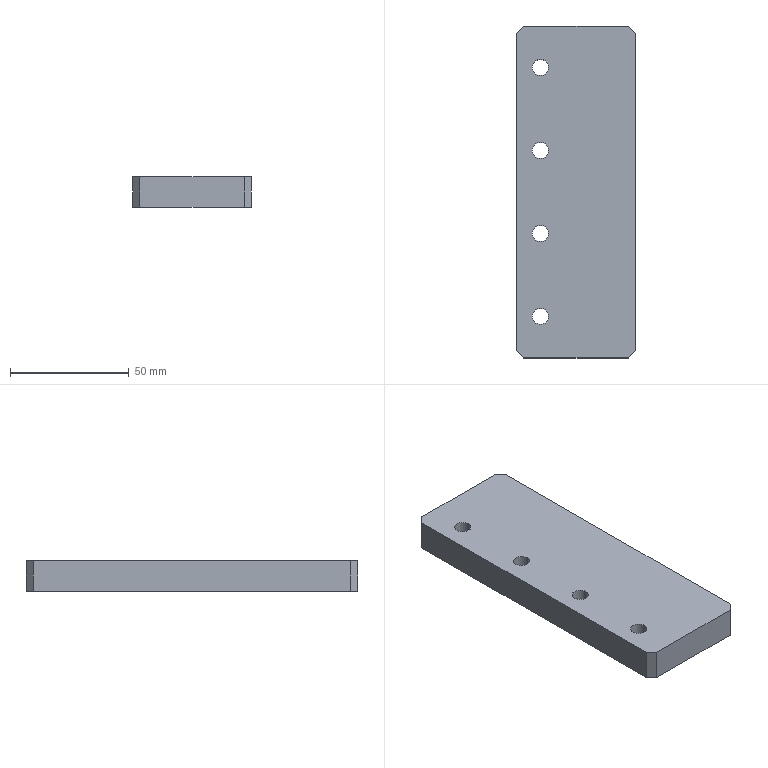Component | SolidWorks | STE21014.01-41-1 | 1 solid | 18 faces | box 50 x 140 x 13 mm | volume 88878 mm3 | plane 10 | cylinder 8 | commonest cylinder face diameters 6.8 x8 | material Q235
build123d program:
from build123d import *

# Parameters (mm, degrees)
SKETCH1_W           = 140
SKETCH1_H           = 50
BOSS_EXTRUDE1_DEPTH = 13
M8_TAPPED_HOLE1_D   = 6.8
CHAMFER1_SIZE       = 3


with BuildPart() as part:
    # Sketch1 → Boss-Extrude1 (new body)
    with BuildSketch(Plane(origin=(0, 0, 0), x_dir=(1, 0, 0), z_dir=(0, 1, 0))):
        Rectangle(SKETCH1_W, SKETCH1_H)
    extrude(amount=BOSS_EXTRUDE1_DEPTH)

    # M8 Tapped Hole1 (through all)
    with Locations(Plane(origin=(0, 13, 0), x_dir=(1, 0, 0), z_dir=(0, 1, 0))):
        with Locations((-52.5, -15), (-17.5, -15), (17.5, -15), (52.5, -15)):
            Hole(M8_TAPPED_HOLE1_D / 2)

    # Chamfer1
    chamfer1_edges = [part.edges().sort_by_distance(p)[0] for p in [
        (-70, 6.5, -25),
        (70, 6.5, -25),
        (70, 6.5, 25),
        (-70, 6.5, 25),
    ]]
    chamfer(chamfer1_edges, length=CHAMFER1_SIZE)


solid = part.part

# Placed as in the assembly
solid = solid.moved(Location((615, 550, -623), (90, -90, 0)))
STEP:
#1=COLOUR_RGB('',0.7922,0.8196,0.9333);
#2=FILL_AREA_STYLE_COLOUR('',#1);
#3=FILL_AREA_STYLE('',(#2));
#4=SURFACE_STYLE_FILL_AREA(#3);
#5=SURFACE_SIDE_STYLE('',(#4));
#6=SURFACE_STYLE_USAGE(.BOTH.,#5);
#7=PRESENTATION_STYLE_ASSIGNMENT((#6));
#8=CARTESIAN_POINT('',(23.756,23.72,-24.528));
#9=VERTEX_POINT('',#8);
#10=CARTESIAN_POINT('',(23.488,23.72,-24.528));
#11=VERTEX_POINT('',#10);
#12=CARTESIAN_POINT('',(23.622,23.72,-24.528));
#13=DIRECTION('',(0.,-0.,1.));
#14=DIRECTION('',(-1.,0.,0.));
#15=AXIS2_PLACEMENT_3D('',#12,#13,#14);
#16=CIRCLE('',#15,0.1339);
#17=EDGE_CURVE('',#9,#11,#16,.T.);
#18=ORIENTED_EDGE('',*,*,#17,.F.);
#19=CARTESIAN_POINT('',(23.756,23.72,-24.016));
#20=VERTEX_POINT('',#19);
#21=CARTESIAN_POINT('',(23.756,23.72,-24.016));
#22=DIRECTION('',(0.,-0.,1.));
#23=VECTOR('',#22,39.37);
#24=LINE('',#21,#23);
#25=EDGE_CURVE('',#9,#20,#24,.T.);
#26=ORIENTED_EDGE('',*,*,#25,.T.);
#27=CARTESIAN_POINT('',(23.488,23.72,-24.016));
#28=VERTEX_POINT('',#27);
#29=CARTESIAN_POINT('',(23.622,23.72,-24.016));
#30=DIRECTION('',(0.,-0.,1.));
#31=DIRECTION('',(-1.,0.,0.));
#32=AXIS2_PLACEMENT_3D('',#29,#30,#31);
#33=CIRCLE('',#32,0.1339);
#34=EDGE_CURVE('',#20,#28,#33,.T.);
#35=ORIENTED_EDGE('',*,*,#34,.T.);
#36=CARTESIAN_POINT('',(23.488,23.72,-24.016));
#37=DIRECTION('',(0.,-0.,1.));
#38=VECTOR('',#37,39.37);
#39=LINE('',#36,#38);
#40=EDGE_CURVE('',#11,#28,#39,.T.);
#41=ORIENTED_EDGE('',*,*,#40,.F.);
#42=EDGE_LOOP('',(#18,#26,#35,#41));
#43=FACE_OUTER_BOUND('',#42,.T.);
#44=CARTESIAN_POINT('',(23.622,23.72,-24.016));
#45=DIRECTION('',(0.,-0.,1.));
#46=DIRECTION('',(-1.,0.,0.));
#47=AXIS2_PLACEMENT_3D('',#44,#45,#46);
#48=CYLINDRICAL_SURFACE('',#47,0.1339);
#49=ADVANCED_FACE('',(#43),#48,.F.);
#50=CARTESIAN_POINT('',(23.756,22.343,-24.528));
#51=VERTEX_POINT('',#50);
#52=CARTESIAN_POINT('',(23.488,22.343,-24.528));
#53=VERTEX_POINT('',#52);
#54=CARTESIAN_POINT('',(23.622,22.343,-24.528));
#55=DIRECTION('',(0.,-0.,1.));
#56=DIRECTION('',(-1.,0.,0.));
#57=AXIS2_PLACEMENT_3D('',#54,#55,#56);
#58=CIRCLE('',#57,0.1339);
#59=EDGE_CURVE('',#51,#53,#58,.T.);
#60=ORIENTED_EDGE('',*,*,#59,.F.);
#61=CARTESIAN_POINT('',(23.756,22.343,-24.016));
#62=VERTEX_POINT('',#61);
#63=CARTESIAN_POINT('',(23.756,22.343,-24.016));
#64=DIRECTION('',(0.,-0.,1.));
#65=VECTOR('',#64,39.37);
#66=LINE('',#63,#65);
#67=EDGE_CURVE('',#51,#62,#66,.T.);
#68=ORIENTED_EDGE('',*,*,#67,.T.);
#69=CARTESIAN_POINT('',(23.488,22.343,-24.016));
#70=VERTEX_POINT('',#69);
#71=CARTESIAN_POINT('',(23.622,22.343,-24.016));
#72=DIRECTION('',(0.,-0.,1.));
#73=DIRECTION('',(-1.,0.,0.));
#74=AXIS2_PLACEMENT_3D('',#71,#72,#73);
#75=CIRCLE('',#74,0.1339);
#76=EDGE_CURVE('',#62,#70,#75,.T.);
#77=ORIENTED_EDGE('',*,*,#76,.T.);
#78=CARTESIAN_POINT('',(23.488,22.343,-24.016));
#79=DIRECTION('',(0.,-0.,1.));
#80=VECTOR('',#79,39.37);
#81=LINE('',#78,#80);
#82=EDGE_CURVE('',#53,#70,#81,.T.);
#83=ORIENTED_EDGE('',*,*,#82,.F.);
#84=EDGE_LOOP('',(#60,#68,#77,#83));
#85=FACE_OUTER_BOUND('',#84,.T.);
#86=CARTESIAN_POINT('',(23.622,22.343,-24.016));
#87=DIRECTION('',(0.,-0.,1.));
#88=DIRECTION('',(-1.,0.,0.));
#89=AXIS2_PLACEMENT_3D('',#86,#87,#88);
#90=CYLINDRICAL_SURFACE('',#89,0.1339);
#91=ADVANCED_FACE('',(#85),#90,.F.);
#92=CARTESIAN_POINT('',(23.756,20.965,-24.528));
#93=VERTEX_POINT('',#92);
#94=CARTESIAN_POINT('',(23.488,20.965,-24.528));
#95=VERTEX_POINT('',#94);
#96=CARTESIAN_POINT('',(23.622,20.965,-24.528));
#97=DIRECTION('',(0.,-0.,1.));
#98=DIRECTION('',(-1.,0.,0.));
#99=AXIS2_PLACEMENT_3D('',#96,#97,#98);
#100=CIRCLE('',#99,0.1339);
#101=EDGE_CURVE('',#93,#95,#100,.T.);
#102=ORIENTED_EDGE('',*,*,#101,.F.);
#103=CARTESIAN_POINT('',(23.756,20.965,-24.016));
#104=VERTEX_POINT('',#103);
#105=CARTESIAN_POINT('',(23.756,20.965,-24.016));
#106=DIRECTION('',(0.,-0.,1.));
#107=VECTOR('',#106,39.37);
#108=LINE('',#105,#107);
#109=EDGE_CURVE('',#93,#104,#108,.T.);
#110=ORIENTED_EDGE('',*,*,#109,.T.);
#111=CARTESIAN_POINT('',(23.488,20.965,-24.016));
#112=VERTEX_POINT('',#111);
#113=CARTESIAN_POINT('',(23.622,20.965,-24.016));
#114=DIRECTION('',(0.,-0.,1.));
#115=DIRECTION('',(-1.,0.,0.));
#116=AXIS2_PLACEMENT_3D('',#113,#114,#115);
#117=CIRCLE('',#116,0.1339);
#118=EDGE_CURVE('',#104,#112,#117,.T.);
#119=ORIENTED_EDGE('',*,*,#118,.T.);
#120=CARTESIAN_POINT('',(23.488,20.965,-24.016));
#121=DIRECTION('',(0.,-0.,1.));
#122=VECTOR('',#121,39.37);
#123=LINE('',#120,#122);
#124=EDGE_CURVE('',#95,#112,#123,.T.);
#125=ORIENTED_EDGE('',*,*,#124,.F.);
#126=EDGE_LOOP('',(#102,#110,#119,#125));
#127=FACE_OUTER_BOUND('',#126,.T.);
#128=CARTESIAN_POINT('',(23.622,20.965,-24.016));
#129=DIRECTION('',(0.,-0.,1.));
#130=DIRECTION('',(-1.,0.,0.));
#131=AXIS2_PLACEMENT_3D('',#128,#129,#130);
#132=CYLINDRICAL_SURFACE('',#131,0.1339);
#133=ADVANCED_FACE('',(#127),#132,.F.);
#134=CARTESIAN_POINT('',(23.756,19.587,-24.528));
#135=VERTEX_POINT('',#134);
#136=CARTESIAN_POINT('',(23.488,19.587,-24.528));
#137=VERTEX_POINT('',#136);
#138=CARTESIAN_POINT('',(23.622,19.587,-24.528));
#139=DIRECTION('',(0.,-0.,1.));
#140=DIRECTION('',(-1.,0.,0.));
#141=AXIS2_PLACEMENT_3D('',#138,#139,#140);
#142=CIRCLE('',#141,0.1339);
#143=EDGE_CURVE('',#135,#137,#142,.T.);
#144=ORIENTED_EDGE('',*,*,#143,.F.);
#145=CARTESIAN_POINT('',(23.756,19.587,-24.016));
#146=VERTEX_POINT('',#145);
#147=CARTESIAN_POINT('',(23.756,19.587,-24.016));
#148=DIRECTION('',(0.,-0.,1.));
#149=VECTOR('',#148,39.37);
#150=LINE('',#147,#149);
#151=EDGE_CURVE('',#135,#146,#150,.T.);
#152=ORIENTED_EDGE('',*,*,#151,.T.);
#153=CARTESIAN_POINT('',(23.488,19.587,-24.016));
#154=VERTEX_POINT('',#153);
#155=CARTESIAN_POINT('',(23.622,19.587,-24.016));
#156=DIRECTION('',(0.,-0.,1.));
#157=DIRECTION('',(-1.,0.,0.));
#158=AXIS2_PLACEMENT_3D('',#155,#156,#157);
#159=CIRCLE('',#158,0.1339);
#160=EDGE_CURVE('',#146,#154,#159,.T.);
#161=ORIENTED_EDGE('',*,*,#160,.T.);
#162=CARTESIAN_POINT('',(23.488,19.587,-24.016));
#163=DIRECTION('',(0.,-0.,1.));
#164=VECTOR('',#163,39.37);
#165=LINE('',#162,#164);
#166=EDGE_CURVE('',#137,#154,#165,.T.);
#167=ORIENTED_EDGE('',*,*,#166,.F.);
#168=EDGE_LOOP('',(#144,#152,#161,#167));
#169=FACE_OUTER_BOUND('',#168,.T.);
#170=CARTESIAN_POINT('',(23.622,19.587,-24.016));
#171=DIRECTION('',(0.,-0.,1.));
#172=DIRECTION('',(-1.,0.,0.));
#173=AXIS2_PLACEMENT_3D('',#170,#171,#172);
#174=CYLINDRICAL_SURFACE('',#173,0.1339);
#175=ADVANCED_FACE('',(#169),#174,.F.);
#176=CARTESIAN_POINT('',(25.079,24.409,-24.016));
#177=VERTEX_POINT('',#176);
#178=CARTESIAN_POINT('',(23.346,24.409,-24.016));
#179=VERTEX_POINT('',#178);
#180=CARTESIAN_POINT('',(23.228,24.409,-24.016));
#181=DIRECTION('',(-1.,0.,0.));
#182=VECTOR('',#181,39.37);
#183=LINE('',#180,#182);
#184=EDGE_CURVE('',#177,#179,#183,.T.);
#185=ORIENTED_EDGE('',*,*,#184,.F.);
#186=CARTESIAN_POINT('',(25.079,24.409,-24.528));
#187=VERTEX_POINT('',#186);
#188=CARTESIAN_POINT('',(25.079,24.409,-24.016));
#189=DIRECTION('',(-0.,0.,-1.));
#190=VECTOR('',#189,39.37);
#191=LINE('',#188,#190);
#192=EDGE_CURVE('',#177,#187,#191,.T.);
#193=ORIENTED_EDGE('',*,*,#192,.T.);
#194=CARTESIAN_POINT('',(23.346,24.409,-24.528));
#195=VERTEX_POINT('',#194);
#196=CARTESIAN_POINT('',(23.228,24.409,-24.528));
#197=DIRECTION('',(-1.,0.,0.));
#198=VECTOR('',#197,39.37);
#199=LINE('',#196,#198);
#200=EDGE_CURVE('',#187,#195,#199,.T.);
#201=ORIENTED_EDGE('',*,*,#200,.T.);
#202=CARTESIAN_POINT('',(23.346,24.409,-24.016));
#203=DIRECTION('',(0.,-0.,1.));
#204=VECTOR('',#203,39.37);
#205=LINE('',#202,#204);
#206=EDGE_CURVE('',#195,#179,#205,.T.);
#207=ORIENTED_EDGE('',*,*,#206,.T.);
#208=EDGE_LOOP('',(#185,#193,#201,#207));
#209=FACE_OUTER_BOUND('',#208,.T.);
#210=CARTESIAN_POINT('',(23.228,24.409,-24.016));
#211=DIRECTION('',(-0.,-1.,-0.));
#212=DIRECTION('',(1.,-0.,-0.));
#213=AXIS2_PLACEMENT_3D('',#210,#211,#212);
#214=PLANE('',#213);
#215=ADVANCED_FACE('',(#209),#214,.F.);
#216=CARTESIAN_POINT('',(23.228,24.291,-24.528));
#217=VERTEX_POINT('',#216);
#218=CARTESIAN_POINT('',(23.228,19.016,-24.528));
#219=VERTEX_POINT('',#218);
#220=CARTESIAN_POINT('',(23.228,18.898,-24.528));
#221=DIRECTION('',(0.,-1.,-0.));
#222=VECTOR('',#221,39.37);
#223=LINE('',#220,#222);
#224=EDGE_CURVE('',#217,#219,#223,.T.);
#225=ORIENTED_EDGE('',*,*,#224,.T.);
#226=CARTESIAN_POINT('',(23.228,19.016,-24.016));
#227=VERTEX_POINT('',#226);
#228=CARTESIAN_POINT('',(23.228,19.016,-24.016));
#229=DIRECTION('',(0.,-0.,1.));
#230=VECTOR('',#229,39.37);
#231=LINE('',#228,#230);
#232=EDGE_CURVE('',#219,#227,#231,.T.);
#233=ORIENTED_EDGE('',*,*,#232,.T.);
#234=CARTESIAN_POINT('',(23.228,24.291,-24.016));
#235=VERTEX_POINT('',#234);
#236=CARTESIAN_POINT('',(23.228,18.898,-24.016));
#237=DIRECTION('',(0.,-1.,-0.));
#238=VECTOR('',#237,39.37);
#239=LINE('',#236,#238);
#240=EDGE_CURVE('',#235,#227,#239,.T.);
#241=ORIENTED_EDGE('',*,*,#240,.F.);
#242=CARTESIAN_POINT('',(23.228,24.291,-24.016));
#243=DIRECTION('',(-0.,0.,-1.));
#244=VECTOR('',#243,39.37);
#245=LINE('',#242,#244);
#246=EDGE_CURVE('',#235,#217,#245,.T.);
#247=ORIENTED_EDGE('',*,*,#246,.T.);
#248=EDGE_LOOP('',(#225,#233,#241,#247));
#249=FACE_OUTER_BOUND('',#248,.T.);
#250=CARTESIAN_POINT('',(23.228,18.898,-24.016));
#251=DIRECTION('',(1.,0.,-0.));
#252=DIRECTION('',(-0.,1.,0.));
#253=AXIS2_PLACEMENT_3D('',#250,#251,#252);
#254=PLANE('',#253);
#255=ADVANCED_FACE('',(#249),#254,.F.);
#256=CARTESIAN_POINT('',(23.346,18.898,-24.016));
#257=VERTEX_POINT('',#256);
#258=CARTESIAN_POINT('',(25.079,18.898,-24.016));
#259=VERTEX_POINT('',#258);
#260=CARTESIAN_POINT('',(23.228,18.898,-24.016));
#261=DIRECTION('',(1.,-0.,-0.));
#262=VECTOR('',#261,39.37);
#263=LINE('',#260,#262);
#264=EDGE_CURVE('',#257,#259,#263,.T.);
#265=ORIENTED_EDGE('',*,*,#264,.F.);
#266=CARTESIAN_POINT('',(23.346,18.898,-24.528));
#267=VERTEX_POINT('',#266);
#268=CARTESIAN_POINT('',(23.346,18.898,-24.016));
#269=DIRECTION('',(-0.,0.,-1.));
#270=VECTOR('',#269,39.37);
#271=LINE('',#268,#270);
#272=EDGE_CURVE('',#257,#267,#271,.T.);
#273=ORIENTED_EDGE('',*,*,#272,.T.);
#274=CARTESIAN_POINT('',(25.079,18.898,-24.528));
#275=VERTEX_POINT('',#274);
#276=CARTESIAN_POINT('',(23.228,18.898,-24.528));
#277=DIRECTION('',(1.,-0.,-0.));
#278=VECTOR('',#277,39.37);
#279=LINE('',#276,#278);
#280=EDGE_CURVE('',#267,#275,#279,.T.);
#281=ORIENTED_EDGE('',*,*,#280,.T.);
#282=CARTESIAN_POINT('',(25.079,18.898,-24.016));
#283=DIRECTION('',(0.,-0.,1.));
#284=VECTOR('',#283,39.37);
#285=LINE('',#282,#284);
#286=EDGE_CURVE('',#275,#259,#285,.T.);
#287=ORIENTED_EDGE('',*,*,#286,.T.);
#288=EDGE_LOOP('',(#265,#273,#281,#287));
#289=FACE_OUTER_BOUND('',#288,.T.);
#290=CARTESIAN_POINT('',(23.228,18.898,-24.016));
#291=DIRECTION('',(0.,1.,0.));
#292=DIRECTION('',(-1.,0.,0.));
#293=AXIS2_PLACEMENT_3D('',#290,#291,#292);
#294=PLANE('',#293);
#295=ADVANCED_FACE('',(#289),#294,.F.);
#296=CARTESIAN_POINT('',(25.197,19.016,-24.016));
#297=VERTEX_POINT('',#296);
#298=CARTESIAN_POINT('',(25.197,24.291,-24.016));
#299=VERTEX_POINT('',#298);
#300=CARTESIAN_POINT('',(25.197,18.898,-24.016));
#301=DIRECTION('',(-0.,1.,0.));
#302=VECTOR('',#301,39.37);
#303=LINE('',#300,#302);
#304=EDGE_CURVE('',#297,#299,#303,.T.);
#305=ORIENTED_EDGE('',*,*,#304,.F.);
#306=CARTESIAN_POINT('',(25.197,19.016,-24.528));
#307=VERTEX_POINT('',#306);
#308=CARTESIAN_POINT('',(25.197,19.016,-24.016));
#309=DIRECTION('',(-0.,0.,-1.));
#310=VECTOR('',#309,39.37);
#311=LINE('',#308,#310);
#312=EDGE_CURVE('',#297,#307,#311,.T.);
#313=ORIENTED_EDGE('',*,*,#312,.T.);
#314=CARTESIAN_POINT('',(25.197,24.291,-24.528));
#315=VERTEX_POINT('',#314);
#316=CARTESIAN_POINT('',(25.197,18.898,-24.528));
#317=DIRECTION('',(-0.,1.,0.));
#318=VECTOR('',#317,39.37);
#319=LINE('',#316,#318);
#320=EDGE_CURVE('',#307,#315,#319,.T.);
#321=ORIENTED_EDGE('',*,*,#320,.T.);
#322=CARTESIAN_POINT('',(25.197,24.291,-24.016));
#323=DIRECTION('',(0.,-0.,1.));
#324=VECTOR('',#323,39.37);
#325=LINE('',#322,#324);
#326=EDGE_CURVE('',#315,#299,#325,.T.);
#327=ORIENTED_EDGE('',*,*,#326,.T.);
#328=EDGE_LOOP('',(#305,#313,#321,#327));
#329=FACE_OUTER_BOUND('',#328,.T.);
#330=CARTESIAN_POINT('',(25.197,18.898,-24.016));
#331=DIRECTION('',(-1.,-0.,0.));
#332=DIRECTION('',(0.,-1.,-0.));
#333=AXIS2_PLACEMENT_3D('',#330,#331,#332);
#334=PLANE('',#333);
#335=ADVANCED_FACE('',(#329),#334,.F.);
#336=CARTESIAN_POINT('',(23.622,23.72,-24.016));
#337=DIRECTION('',(0.,-0.,1.));
#338=DIRECTION('',(-1.,0.,0.));
#339=AXIS2_PLACEMENT_3D('',#336,#337,#338);
#340=CIRCLE('',#339,0.1339);
#341=EDGE_CURVE('',#28,#20,#340,.T.);
#342=ORIENTED_EDGE('',*,*,#341,.F.);
#343=ORIENTED_EDGE('',*,*,#34,.F.);
#344=EDGE_LOOP('',(#342,#343));
#345=FACE_BOUND('',#344,.T.);
#346=CARTESIAN_POINT('',(23.622,22.343,-24.016));
#347=DIRECTION('',(0.,-0.,1.));
#348=DIRECTION('',(-1.,0.,0.));
#349=AXIS2_PLACEMENT_3D('',#346,#347,#348);
#350=CIRCLE('',#349,0.1339);
#351=EDGE_CURVE('',#70,#62,#350,.T.);
#352=ORIENTED_EDGE('',*,*,#351,.F.);
#353=ORIENTED_EDGE('',*,*,#76,.F.);
#354=EDGE_LOOP('',(#352,#353));
#355=FACE_BOUND('',#354,.T.);
#356=CARTESIAN_POINT('',(23.622,20.965,-24.016));
#357=DIRECTION('',(0.,-0.,1.));
#358=DIRECTION('',(-1.,0.,0.));
#359=AXIS2_PLACEMENT_3D('',#356,#357,#358);
#360=CIRCLE('',#359,0.1339);
#361=EDGE_CURVE('',#112,#104,#360,.T.);
#362=ORIENTED_EDGE('',*,*,#361,.F.);
#363=ORIENTED_EDGE('',*,*,#118,.F.);
#364=EDGE_LOOP('',(#362,#363));
#365=FACE_BOUND('',#364,.T.);
#366=CARTESIAN_POINT('',(23.622,19.587,-24.016));
#367=DIRECTION('',(0.,-0.,1.));
#368=DIRECTION('',(-1.,0.,0.));
#369=AXIS2_PLACEMENT_3D('',#366,#367,#368);
#370=CIRCLE('',#369,0.1339);
#371=EDGE_CURVE('',#154,#146,#370,.T.);
#372=ORIENTED_EDGE('',*,*,#371,.F.);
#373=ORIENTED_EDGE('',*,*,#160,.F.);
#374=EDGE_LOOP('',(#372,#373));
#375=FACE_BOUND('',#374,.T.);
#376=ORIENTED_EDGE('',*,*,#240,.T.);
#377=CARTESIAN_POINT('',(22.402,19.843,-24.016));
#378=DIRECTION('',(0.7071,-0.7071,-0.));
#379=VECTOR('',#378,39.37);
#380=LINE('',#377,#379);
#381=EDGE_CURVE('',#227,#257,#380,.T.);
#382=ORIENTED_EDGE('',*,*,#381,.T.);
#383=ORIENTED_EDGE('',*,*,#264,.T.);
#384=CARTESIAN_POINT('',(26.024,19.843,-24.016));
#385=DIRECTION('',(0.7071,0.7071,0.));
#386=VECTOR('',#385,39.37);
#387=LINE('',#384,#386);
#388=EDGE_CURVE('',#259,#297,#387,.T.);
#389=ORIENTED_EDGE('',*,*,#388,.T.);
#390=ORIENTED_EDGE('',*,*,#304,.T.);
#391=CARTESIAN_POINT('',(26.024,23.465,-24.016));
#392=DIRECTION('',(-0.7071,0.7071,0.));
#393=VECTOR('',#392,39.37);
#394=LINE('',#391,#393);
#395=EDGE_CURVE('',#299,#177,#394,.T.);
#396=ORIENTED_EDGE('',*,*,#395,.T.);
#397=ORIENTED_EDGE('',*,*,#184,.T.);
#398=CARTESIAN_POINT('',(22.402,23.465,-24.016));
#399=DIRECTION('',(-0.7071,-0.7071,-0.));
#400=VECTOR('',#399,39.37);
#401=LINE('',#398,#400);
#402=EDGE_CURVE('',#179,#235,#401,.T.);
#403=ORIENTED_EDGE('',*,*,#402,.T.);
#404=EDGE_LOOP('',(#376,#382,#383,#389,#390,#396,#397,#403));
#405=FACE_OUTER_BOUND('',#404,.T.);
#406=CARTESIAN_POINT('',(24.213,21.654,-24.016));
#407=DIRECTION('',(0.,-0.,1.));
#408=DIRECTION('',(-1.,0.,0.));
#409=AXIS2_PLACEMENT_3D('',#406,#407,#408);
#410=PLANE('',#409);
#411=ADVANCED_FACE('',(#345,#355,#365,#375,#405),#410,.T.);
#412=CARTESIAN_POINT('',(23.622,23.72,-24.528));
#413=DIRECTION('',(0.,-0.,1.));
#414=DIRECTION('',(-1.,0.,0.));
#415=AXIS2_PLACEMENT_3D('',#412,#413,#414);
#416=CIRCLE('',#415,0.1339);
#417=EDGE_CURVE('',#11,#9,#416,.T.);
#418=ORIENTED_EDGE('',*,*,#417,.T.);
#419=ORIENTED_EDGE('',*,*,#17,.T.);
#420=EDGE_LOOP('',(#418,#419));
#421=FACE_BOUND('',#420,.T.);
#422=CARTESIAN_POINT('',(23.622,22.343,-24.528));
#423=DIRECTION('',(0.,-0.,1.));
#424=DIRECTION('',(-1.,0.,0.));
#425=AXIS2_PLACEMENT_3D('',#422,#423,#424);
#426=CIRCLE('',#425,0.1339);
#427=EDGE_CURVE('',#53,#51,#426,.T.);
#428=ORIENTED_EDGE('',*,*,#427,.T.);
#429=ORIENTED_EDGE('',*,*,#59,.T.);
#430=EDGE_LOOP('',(#428,#429));
#431=FACE_BOUND('',#430,.T.);
#432=CARTESIAN_POINT('',(23.622,20.965,-24.528));
#433=DIRECTION('',(0.,-0.,1.));
#434=DIRECTION('',(-1.,0.,0.));
#435=AXIS2_PLACEMENT_3D('',#432,#433,#434);
#436=CIRCLE('',#435,0.1339);
#437=EDGE_CURVE('',#95,#93,#436,.T.);
#438=ORIENTED_EDGE('',*,*,#437,.T.);
#439=ORIENTED_EDGE('',*,*,#101,.T.);
#440=EDGE_LOOP('',(#438,#439));
#441=FACE_BOUND('',#440,.T.);
#442=CARTESIAN_POINT('',(23.622,19.587,-24.528));
#443=DIRECTION('',(0.,-0.,1.));
#444=DIRECTION('',(-1.,0.,0.));
#445=AXIS2_PLACEMENT_3D('',#442,#443,#444);
#446=CIRCLE('',#445,0.1339);
#447=EDGE_CURVE('',#137,#135,#446,.T.);
#448=ORIENTED_EDGE('',*,*,#447,.T.);
#449=ORIENTED_EDGE('',*,*,#143,.T.);
#450=EDGE_LOOP('',(#448,#449));
#451=FACE_BOUND('',#450,.T.);
#452=ORIENTED_EDGE('',*,*,#280,.F.);
#453=CARTESIAN_POINT('',(23.346,18.898,-24.528));
#454=DIRECTION('',(-0.7071,0.7071,0.));
#455=VECTOR('',#454,39.37);
#456=LINE('',#453,#455);
#457=EDGE_CURVE('',#267,#219,#456,.T.);
#458=ORIENTED_EDGE('',*,*,#457,.T.);
#459=ORIENTED_EDGE('',*,*,#224,.F.);
#460=CARTESIAN_POINT('',(23.228,24.291,-24.528));
#461=DIRECTION('',(0.7071,0.7071,0.));
#462=VECTOR('',#461,39.37);
#463=LINE('',#460,#462);
#464=EDGE_CURVE('',#217,#195,#463,.T.);
#465=ORIENTED_EDGE('',*,*,#464,.T.);
#466=ORIENTED_EDGE('',*,*,#200,.F.);
#467=CARTESIAN_POINT('',(25.079,24.409,-24.528));
#468=DIRECTION('',(0.7071,-0.7071,-0.));
#469=VECTOR('',#468,39.37);
#470=LINE('',#467,#469);
#471=EDGE_CURVE('',#187,#315,#470,.T.);
#472=ORIENTED_EDGE('',*,*,#471,.T.);
#473=ORIENTED_EDGE('',*,*,#320,.F.);
#474=CARTESIAN_POINT('',(25.197,19.016,-24.528));
#475=DIRECTION('',(-0.7071,-0.7071,-0.));
#476=VECTOR('',#475,39.37);
#477=LINE('',#474,#476);
#478=EDGE_CURVE('',#307,#275,#477,.T.);
#479=ORIENTED_EDGE('',*,*,#478,.T.);
#480=EDGE_LOOP('',(#452,#458,#459,#465,#466,#472,#473,#479));
#481=FACE_OUTER_BOUND('',#480,.T.);
#482=CARTESIAN_POINT('',(24.213,21.654,-24.528));
#483=DIRECTION('',(0.,-0.,1.));
#484=DIRECTION('',(-1.,0.,0.));
#485=AXIS2_PLACEMENT_3D('',#482,#483,#484);
#486=PLANE('',#485);
#487=ADVANCED_FACE('',(#421,#431,#441,#451,#481),#486,.F.);
#488=ORIENTED_EDGE('',*,*,#151,.F.);
#489=ORIENTED_EDGE('',*,*,#447,.F.);
#490=ORIENTED_EDGE('',*,*,#166,.T.);
#491=ORIENTED_EDGE('',*,*,#371,.T.);
#492=EDGE_LOOP('',(#488,#489,#490,#491));
#493=FACE_OUTER_BOUND('',#492,.T.);
#494=CARTESIAN_POINT('',(23.622,19.587,-24.016));
#495=DIRECTION('',(0.,-0.,1.));
#496=DIRECTION('',(-1.,0.,0.));
#497=AXIS2_PLACEMENT_3D('',#494,#495,#496);
#498=CYLINDRICAL_SURFACE('',#497,0.1339);
#499=ADVANCED_FACE('',(#493),#498,.F.);
#500=ORIENTED_EDGE('',*,*,#109,.F.);
#501=ORIENTED_EDGE('',*,*,#437,.F.);
#502=ORIENTED_EDGE('',*,*,#124,.T.);
#503=ORIENTED_EDGE('',*,*,#361,.T.);
#504=EDGE_LOOP('',(#500,#501,#502,#503));
#505=FACE_OUTER_BOUND('',#504,.T.);
#506=CARTESIAN_POINT('',(23.622,20.965,-24.016));
#507=DIRECTION('',(0.,-0.,1.));
#508=DIRECTION('',(-1.,0.,0.));
#509=AXIS2_PLACEMENT_3D('',#506,#507,#508);
#510=CYLINDRICAL_SURFACE('',#509,0.1339);
#511=ADVANCED_FACE('',(#505),#510,.F.);
#512=ORIENTED_EDGE('',*,*,#67,.F.);
#513=ORIENTED_EDGE('',*,*,#427,.F.);
#514=ORIENTED_EDGE('',*,*,#82,.T.);
#515=ORIENTED_EDGE('',*,*,#351,.T.);
#516=EDGE_LOOP('',(#512,#513,#514,#515));
#517=FACE_OUTER_BOUND('',#516,.T.);
#518=CARTESIAN_POINT('',(23.622,22.343,-24.016));
#519=DIRECTION('',(0.,-0.,1.));
#520=DIRECTION('',(-1.,0.,0.));
#521=AXIS2_PLACEMENT_3D('',#518,#519,#520);
#522=CYLINDRICAL_SURFACE('',#521,0.1339);
#523=ADVANCED_FACE('',(#517),#522,.F.);
#524=ORIENTED_EDGE('',*,*,#25,.F.);
#525=ORIENTED_EDGE('',*,*,#417,.F.);
#526=ORIENTED_EDGE('',*,*,#40,.T.);
#527=ORIENTED_EDGE('',*,*,#341,.T.);
#528=EDGE_LOOP('',(#524,#525,#526,#527));
#529=FACE_OUTER_BOUND('',#528,.T.);
#530=CARTESIAN_POINT('',(23.622,23.72,-24.016));
#531=DIRECTION('',(0.,-0.,1.));
#532=DIRECTION('',(-1.,0.,0.));
#533=AXIS2_PLACEMENT_3D('',#530,#531,#532);
#534=CYLINDRICAL_SURFACE('',#533,0.1339);
#535=ADVANCED_FACE('',(#529),#534,.F.);
#536=ORIENTED_EDGE('',*,*,#381,.F.);
#537=ORIENTED_EDGE('',*,*,#232,.F.);
#538=ORIENTED_EDGE('',*,*,#457,.F.);
#539=ORIENTED_EDGE('',*,*,#272,.F.);
#540=EDGE_LOOP('',(#536,#537,#538,#539));
#541=FACE_OUTER_BOUND('',#540,.T.);
#542=CARTESIAN_POINT('',(23.346,18.898,-24.016));
#543=DIRECTION('',(0.7071,0.7071,0.));
#544=DIRECTION('',(-0.,0.,-1.));
#545=AXIS2_PLACEMENT_3D('',#542,#543,#544);
#546=PLANE('',#545);
#547=ADVANCED_FACE('',(#541),#546,.F.);
#548=ORIENTED_EDGE('',*,*,#388,.F.);
#549=ORIENTED_EDGE('',*,*,#286,.F.);
#550=ORIENTED_EDGE('',*,*,#478,.F.);
#551=ORIENTED_EDGE('',*,*,#312,.F.);
#552=EDGE_LOOP('',(#548,#549,#550,#551));
#553=FACE_OUTER_BOUND('',#552,.T.);
#554=CARTESIAN_POINT('',(25.197,19.016,-24.016));
#555=DIRECTION('',(-0.7071,0.7071,0.));
#556=DIRECTION('',(-0.,0.,-1.));
#557=AXIS2_PLACEMENT_3D('',#554,#555,#556);
#558=PLANE('',#557);
#559=ADVANCED_FACE('',(#553),#558,.F.);
#560=ORIENTED_EDGE('',*,*,#395,.F.);
#561=ORIENTED_EDGE('',*,*,#326,.F.);
#562=ORIENTED_EDGE('',*,*,#471,.F.);
#563=ORIENTED_EDGE('',*,*,#192,.F.);
#564=EDGE_LOOP('',(#560,#561,#562,#563));
#565=FACE_OUTER_BOUND('',#564,.T.);
#566=CARTESIAN_POINT('',(25.079,24.409,-24.016));
#567=DIRECTION('',(-0.7071,-0.7071,-0.));
#568=DIRECTION('',(-0.,0.,-1.));
#569=AXIS2_PLACEMENT_3D('',#566,#567,#568);
#570=PLANE('',#569);
#571=ADVANCED_FACE('',(#565),#570,.F.);
#572=ORIENTED_EDGE('',*,*,#402,.F.);
#573=ORIENTED_EDGE('',*,*,#206,.F.);
#574=ORIENTED_EDGE('',*,*,#464,.F.);
#575=ORIENTED_EDGE('',*,*,#246,.F.);
#576=EDGE_LOOP('',(#572,#573,#574,#575));
#577=FACE_OUTER_BOUND('',#576,.T.);
#578=CARTESIAN_POINT('',(23.228,24.291,-24.016));
#579=DIRECTION('',(0.7071,-0.7071,-0.));
#580=DIRECTION('',(-0.,0.,-1.));
#581=AXIS2_PLACEMENT_3D('',#578,#579,#580);
#582=PLANE('',#581);
#583=ADVANCED_FACE('',(#577),#582,.F.);
#584=CLOSED_SHELL('',(#49,#91,#133,#175,#215,#255,#295,#335,#411,#487,#499,#511,#523,#535,#547,#559,#571,#583));
#585=MANIFOLD_SOLID_BREP('',#584);
#586=STYLED_ITEM('',(#7),#585);
#587=(LENGTH_UNIT()NAMED_UNIT(*)SI_UNIT($,.METRE.));
#588=LENGTH_MEASURE_WITH_UNIT(LENGTH_MEASURE(0.0254),#587);
#589=DIMENSIONAL_EXPONENTS(1.,0.,0.,0.,0.,0.,0.);
#590=(CONVERSION_BASED_UNIT('',#588)LENGTH_UNIT()NAMED_UNIT(#589));
#591=UNCERTAINTY_MEASURE_WITH_UNIT(LENGTH_MEASURE(0.00001),#590,'','');
#592=(NAMED_UNIT(*)PLANE_ANGLE_UNIT()SI_UNIT($,.RADIAN.));
#593=(NAMED_UNIT(*)SI_UNIT($,.STERADIAN.)SOLID_ANGLE_UNIT());
#594=(GEOMETRIC_REPRESENTATION_CONTEXT(3)GLOBAL_UNCERTAINTY_ASSIGNED_CONTEXT((#591))GLOBAL_UNIT_ASSIGNED_CONTEXT((#590,#592,#593))REPRESENTATION_CONTEXT('',''));
#595=MECHANICAL_DESIGN_GEOMETRIC_PRESENTATION_REPRESENTATION('',(#586),#594);
#596=PRESENTATION_LAYER_ASSIGNMENT('','',(#586));
#597=CARTESIAN_POINT('',(0.,0.,0.));
#598=DIRECTION('',(0.,0.,1.));
#599=DIRECTION('',(1.,0.,0.));
#600=AXIS2_PLACEMENT_3D('',#597,#598,#599);
#601=(LENGTH_UNIT()NAMED_UNIT(*)SI_UNIT($,.METRE.));
#602=LENGTH_MEASURE_WITH_UNIT(LENGTH_MEASURE(0.0254),#601);
#603=DIMENSIONAL_EXPONENTS(1.,0.,0.,0.,0.,0.,0.);
#604=(CONVERSION_BASED_UNIT('',#602)LENGTH_UNIT()NAMED_UNIT(#603));
#605=UNCERTAINTY_MEASURE_WITH_UNIT(LENGTH_MEASURE(0.00001),#604,'','');
#606=(NAMED_UNIT(*)PLANE_ANGLE_UNIT()SI_UNIT($,.RADIAN.));
#607=(NAMED_UNIT(*)SI_UNIT($,.STERADIAN.)SOLID_ANGLE_UNIT());
#608=(GEOMETRIC_REPRESENTATION_CONTEXT(3)GLOBAL_UNCERTAINTY_ASSIGNED_CONTEXT((#605))GLOBAL_UNIT_ASSIGNED_CONTEXT((#604,#606,#607))REPRESENTATION_CONTEXT('',''));
#609=ADVANCED_BREP_SHAPE_REPRESENTATION('',(#585,#600),#608);